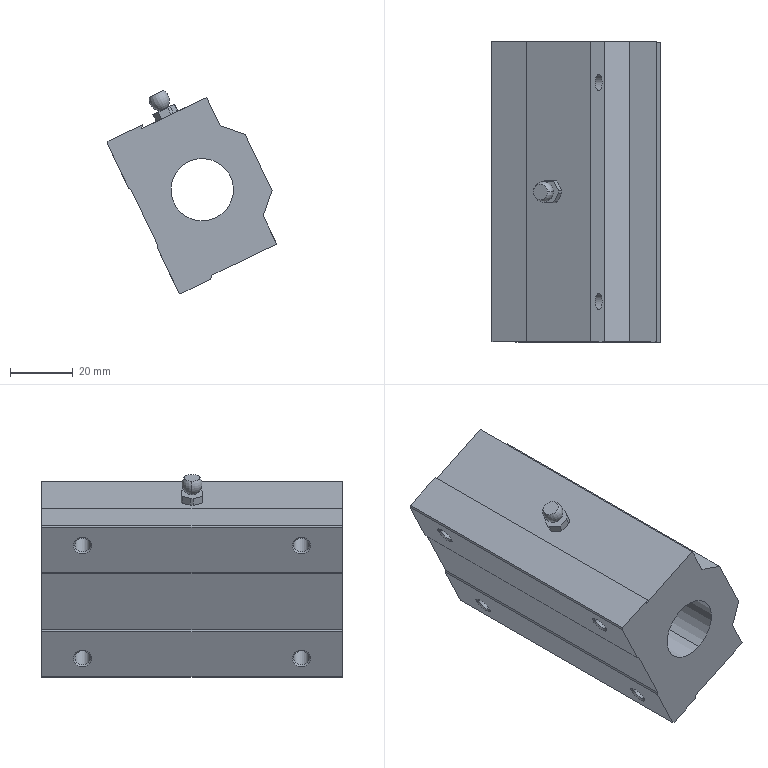Component | SolidWorks | Bearing-1 | 1 solid | 78 faces | volume 158196 mm3 | plane 33 | cone 23 | cylinder 20 | torus 2 | commonest cylinder face diameters 4.917 x8 5.2 x8 8.08 x2 20 x2